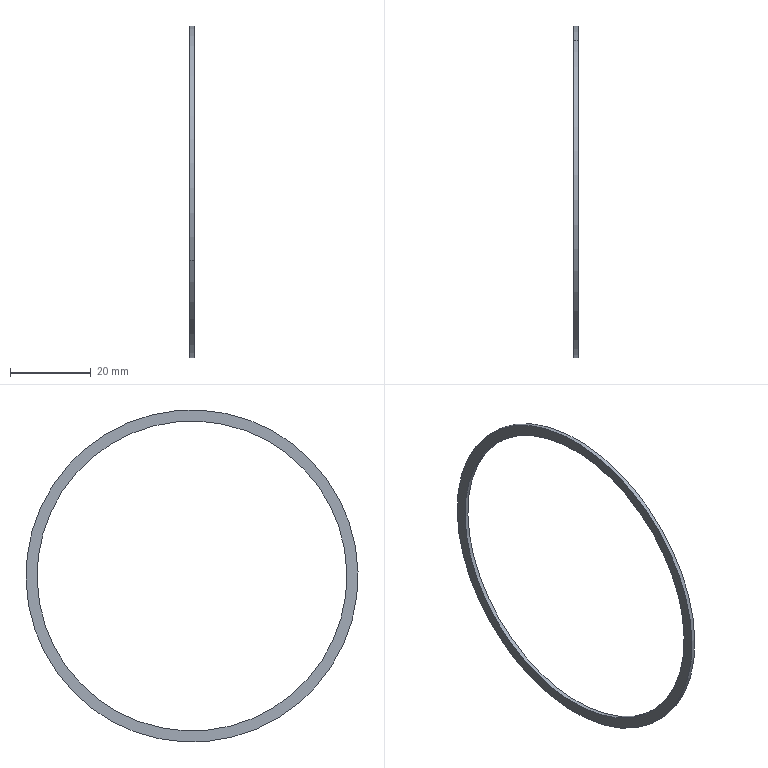Component | SolidWorks | 2018SOLIDWORKS1000000503-1 | 1 solid | 6 faces | box 1 x 82 x 82 mm | volume 685 mm3 | cylinder 4 | plane 2 | commonest cylinder face diameters 76.5 x2 82 x2 | material 201
build123d program:
from build123d import *

# Parameters (mm, degrees)
SKETCH1_R           = 41
SKETCH1_R_2         = 38.25
BOSS_EXTRUDE1_DEPTH = 1


with BuildPart() as part:
    # Sketch1 → Boss-Extrude1 (new body)
    with BuildSketch(Plane.XY):
        Circle(SKETCH1_R)
        Circle(SKETCH1_R_2, mode=Mode.SUBTRACT)
    extrude(amount=BOSS_EXTRUDE1_DEPTH)


solid = part.part

# Placed as in the assembly
solid = solid.moved(Location((6.716, -95.825, 207.018), (0, 90, 0)))
STEP:
#1=COLOUR_RGB('',0.7922,0.8196,0.9333);
#2=FILL_AREA_STYLE_COLOUR('',#1);
#3=FILL_AREA_STYLE('',(#2));
#4=SURFACE_STYLE_FILL_AREA(#3);
#5=SURFACE_SIDE_STYLE('',(#4));
#6=SURFACE_STYLE_USAGE(.BOTH.,#5);
#7=PRESENTATION_STYLE_ASSIGNMENT((#6));
#8=CARTESIAN_POINT('',(0.3038,-5.145,7.53));
#9=VERTEX_POINT('',#8);
#10=CARTESIAN_POINT('',(0.3038,-2.4,8.771));
#11=VERTEX_POINT('',#10);
#12=CARTESIAN_POINT('',(0.3038,-3.773,8.15));
#13=DIRECTION('',(1.,0.,-0.));
#14=DIRECTION('',(-0.,0.9112,0.4119));
#15=AXIS2_PLACEMENT_3D('',#12,#13,#14);
#16=CIRCLE('',#15,1.506);
#17=EDGE_CURVE('',#9,#11,#16,.T.);
#18=ORIENTED_EDGE('',*,*,#17,.T.);
#19=CARTESIAN_POINT('',(0.2644,-2.4,8.771));
#20=VERTEX_POINT('',#19);
#21=CARTESIAN_POINT('',(0.3038,-2.4,8.771));
#22=DIRECTION('',(-1.,-0.,0.));
#23=VECTOR('',#22,39.37);
#24=LINE('',#21,#23);
#25=EDGE_CURVE('',#11,#20,#24,.T.);
#26=ORIENTED_EDGE('',*,*,#25,.T.);
#27=CARTESIAN_POINT('',(0.2644,-5.145,7.53));
#28=VERTEX_POINT('',#27);
#29=CARTESIAN_POINT('',(0.2644,-3.773,8.15));
#30=DIRECTION('',(1.,0.,-0.));
#31=DIRECTION('',(-0.,0.9112,0.4119));
#32=AXIS2_PLACEMENT_3D('',#29,#30,#31);
#33=CIRCLE('',#32,1.506);
#34=EDGE_CURVE('',#28,#20,#33,.T.);
#35=ORIENTED_EDGE('',*,*,#34,.F.);
#36=CARTESIAN_POINT('',(0.3038,-5.145,7.53));
#37=DIRECTION('',(-1.,-0.,0.));
#38=VECTOR('',#37,39.37);
#39=LINE('',#36,#38);
#40=EDGE_CURVE('',#9,#28,#39,.T.);
#41=ORIENTED_EDGE('',*,*,#40,.F.);
#42=EDGE_LOOP('',(#18,#26,#35,#41));
#43=FACE_OUTER_BOUND('',#42,.T.);
#44=CARTESIAN_POINT('',(0.3038,-3.773,8.15));
#45=DIRECTION('',(-1.,-0.,0.));
#46=DIRECTION('',(0.,-0.9112,-0.4119));
#47=AXIS2_PLACEMENT_3D('',#44,#45,#46);
#48=CYLINDRICAL_SURFACE('',#47,1.506);
#49=ADVANCED_FACE('',(#43),#48,.F.);
#50=CARTESIAN_POINT('',(0.3038,-2.302,8.815));
#51=VERTEX_POINT('',#50);
#52=CARTESIAN_POINT('',(0.3038,-5.244,7.485));
#53=VERTEX_POINT('',#52);
#54=CARTESIAN_POINT('',(0.3038,-3.773,8.15));
#55=DIRECTION('',(1.,0.,-0.));
#56=DIRECTION('',(-0.,0.9112,0.4119));
#57=AXIS2_PLACEMENT_3D('',#54,#55,#56);
#58=CIRCLE('',#57,1.614);
#59=EDGE_CURVE('',#51,#53,#58,.T.);
#60=ORIENTED_EDGE('',*,*,#59,.F.);
#61=CARTESIAN_POINT('',(0.2644,-2.302,8.815));
#62=VERTEX_POINT('',#61);
#63=CARTESIAN_POINT('',(0.3038,-2.302,8.815));
#64=DIRECTION('',(-1.,-0.,0.));
#65=VECTOR('',#64,39.37);
#66=LINE('',#63,#65);
#67=EDGE_CURVE('',#51,#62,#66,.T.);
#68=ORIENTED_EDGE('',*,*,#67,.T.);
#69=CARTESIAN_POINT('',(0.2644,-5.244,7.485));
#70=VERTEX_POINT('',#69);
#71=CARTESIAN_POINT('',(0.2644,-3.773,8.15));
#72=DIRECTION('',(1.,0.,-0.));
#73=DIRECTION('',(-0.,0.9112,0.4119));
#74=AXIS2_PLACEMENT_3D('',#71,#72,#73);
#75=CIRCLE('',#74,1.614);
#76=EDGE_CURVE('',#62,#70,#75,.T.);
#77=ORIENTED_EDGE('',*,*,#76,.T.);
#78=CARTESIAN_POINT('',(0.3038,-5.244,7.485));
#79=DIRECTION('',(-1.,-0.,0.));
#80=VECTOR('',#79,39.37);
#81=LINE('',#78,#80);
#82=EDGE_CURVE('',#53,#70,#81,.T.);
#83=ORIENTED_EDGE('',*,*,#82,.F.);
#84=EDGE_LOOP('',(#60,#68,#77,#83));
#85=FACE_OUTER_BOUND('',#84,.T.);
#86=CARTESIAN_POINT('',(0.3038,-3.773,8.15));
#87=DIRECTION('',(-1.,-0.,0.));
#88=DIRECTION('',(0.,-0.9112,-0.4119));
#89=AXIS2_PLACEMENT_3D('',#86,#87,#88);
#90=CYLINDRICAL_SURFACE('',#89,1.614);
#91=ADVANCED_FACE('',(#85),#90,.T.);
#92=CARTESIAN_POINT('',(0.3038,-3.773,8.15));
#93=DIRECTION('',(1.,0.,-0.));
#94=DIRECTION('',(-0.,0.9112,0.4119));
#95=AXIS2_PLACEMENT_3D('',#92,#93,#94);
#96=CIRCLE('',#95,1.614);
#97=EDGE_CURVE('',#53,#51,#96,.T.);
#98=ORIENTED_EDGE('',*,*,#97,.T.);
#99=ORIENTED_EDGE('',*,*,#59,.T.);
#100=EDGE_LOOP('',(#98,#99));
#101=FACE_OUTER_BOUND('',#100,.T.);
#102=ORIENTED_EDGE('',*,*,#17,.F.);
#103=CARTESIAN_POINT('',(0.3038,-3.773,8.15));
#104=DIRECTION('',(1.,0.,-0.));
#105=DIRECTION('',(-0.,0.9112,0.4119));
#106=AXIS2_PLACEMENT_3D('',#103,#104,#105);
#107=CIRCLE('',#106,1.506);
#108=EDGE_CURVE('',#11,#9,#107,.T.);
#109=ORIENTED_EDGE('',*,*,#108,.F.);
#110=EDGE_LOOP('',(#102,#109));
#111=FACE_BOUND('',#110,.T.);
#112=CARTESIAN_POINT('',(0.3038,-3.773,8.15));
#113=DIRECTION('',(1.,0.,-0.));
#114=DIRECTION('',(-0.,0.9112,0.4119));
#115=AXIS2_PLACEMENT_3D('',#112,#113,#114);
#116=PLANE('',#115);
#117=ADVANCED_FACE('',(#101,#111),#116,.T.);
#118=CARTESIAN_POINT('',(0.2644,-3.773,8.15));
#119=DIRECTION('',(1.,0.,-0.));
#120=DIRECTION('',(-0.,0.9112,0.4119));
#121=AXIS2_PLACEMENT_3D('',#118,#119,#120);
#122=CIRCLE('',#121,1.614);
#123=EDGE_CURVE('',#70,#62,#122,.T.);
#124=ORIENTED_EDGE('',*,*,#123,.F.);
#125=ORIENTED_EDGE('',*,*,#76,.F.);
#126=EDGE_LOOP('',(#124,#125));
#127=FACE_OUTER_BOUND('',#126,.T.);
#128=ORIENTED_EDGE('',*,*,#34,.T.);
#129=CARTESIAN_POINT('',(0.2644,-3.773,8.15));
#130=DIRECTION('',(1.,0.,-0.));
#131=DIRECTION('',(-0.,0.9112,0.4119));
#132=AXIS2_PLACEMENT_3D('',#129,#130,#131);
#133=CIRCLE('',#132,1.506);
#134=EDGE_CURVE('',#20,#28,#133,.T.);
#135=ORIENTED_EDGE('',*,*,#134,.T.);
#136=EDGE_LOOP('',(#128,#135));
#137=FACE_BOUND('',#136,.T.);
#138=CARTESIAN_POINT('',(0.2644,-3.773,8.15));
#139=DIRECTION('',(1.,0.,-0.));
#140=DIRECTION('',(-0.,0.9112,0.4119));
#141=AXIS2_PLACEMENT_3D('',#138,#139,#140);
#142=PLANE('',#141);
#143=ADVANCED_FACE('',(#127,#137),#142,.F.);
#144=ORIENTED_EDGE('',*,*,#67,.F.);
#145=ORIENTED_EDGE('',*,*,#97,.F.);
#146=ORIENTED_EDGE('',*,*,#82,.T.);
#147=ORIENTED_EDGE('',*,*,#123,.T.);
#148=EDGE_LOOP('',(#144,#145,#146,#147));
#149=FACE_OUTER_BOUND('',#148,.T.);
#150=CARTESIAN_POINT('',(0.3038,-3.773,8.15));
#151=DIRECTION('',(-1.,-0.,0.));
#152=DIRECTION('',(0.,-0.9112,-0.4119));
#153=AXIS2_PLACEMENT_3D('',#150,#151,#152);
#154=CYLINDRICAL_SURFACE('',#153,1.614);
#155=ADVANCED_FACE('',(#149),#154,.T.);
#156=ORIENTED_EDGE('',*,*,#25,.F.);
#157=ORIENTED_EDGE('',*,*,#108,.T.);
#158=ORIENTED_EDGE('',*,*,#40,.T.);
#159=ORIENTED_EDGE('',*,*,#134,.F.);
#160=EDGE_LOOP('',(#156,#157,#158,#159));
#161=FACE_OUTER_BOUND('',#160,.T.);
#162=CARTESIAN_POINT('',(0.3038,-3.773,8.15));
#163=DIRECTION('',(-1.,-0.,0.));
#164=DIRECTION('',(0.,-0.9112,-0.4119));
#165=AXIS2_PLACEMENT_3D('',#162,#163,#164);
#166=CYLINDRICAL_SURFACE('',#165,1.506);
#167=ADVANCED_FACE('',(#161),#166,.F.);
#168=CLOSED_SHELL('',(#49,#91,#117,#143,#155,#167));
#169=MANIFOLD_SOLID_BREP('',#168);
#170=STYLED_ITEM('',(#7),#169);
#171=PRESENTATION_LAYER_ASSIGNMENT('','',(#170));
#172=(LENGTH_UNIT()NAMED_UNIT(*)SI_UNIT($,.METRE.));
#173=LENGTH_MEASURE_WITH_UNIT(LENGTH_MEASURE(0.0254),#172);
#174=DIMENSIONAL_EXPONENTS(1.,0.,0.,0.,0.,0.,0.);
#175=(CONVERSION_BASED_UNIT('',#173)LENGTH_UNIT()NAMED_UNIT(#174));
#176=UNCERTAINTY_MEASURE_WITH_UNIT(LENGTH_MEASURE(0.00001),#175,'','');
#177=(NAMED_UNIT(*)PLANE_ANGLE_UNIT()SI_UNIT($,.RADIAN.));
#178=(NAMED_UNIT(*)SI_UNIT($,.STERADIAN.)SOLID_ANGLE_UNIT());
#179=(GEOMETRIC_REPRESENTATION_CONTEXT(3)GLOBAL_UNCERTAINTY_ASSIGNED_CONTEXT((#176))GLOBAL_UNIT_ASSIGNED_CONTEXT((#175,#177,#178))REPRESENTATION_CONTEXT('',''));
#180=MECHANICAL_DESIGN_GEOMETRIC_PRESENTATION_REPRESENTATION('',(#170),#179);
#181=CARTESIAN_POINT('',(0.,0.,0.));
#182=DIRECTION('',(0.,0.,1.));
#183=DIRECTION('',(1.,0.,0.));
#184=AXIS2_PLACEMENT_3D('',#181,#182,#183);
#185=(LENGTH_UNIT()NAMED_UNIT(*)SI_UNIT($,.METRE.));
#186=LENGTH_MEASURE_WITH_UNIT(LENGTH_MEASURE(0.0254),#185);
#187=DIMENSIONAL_EXPONENTS(1.,0.,0.,0.,0.,0.,0.);
#188=(CONVERSION_BASED_UNIT('',#186)LENGTH_UNIT()NAMED_UNIT(#187));
#189=UNCERTAINTY_MEASURE_WITH_UNIT(LENGTH_MEASURE(0.00001),#188,'','');
#190=(NAMED_UNIT(*)PLANE_ANGLE_UNIT()SI_UNIT($,.RADIAN.));
#191=(NAMED_UNIT(*)SI_UNIT($,.STERADIAN.)SOLID_ANGLE_UNIT());
#192=(GEOMETRIC_REPRESENTATION_CONTEXT(3)GLOBAL_UNCERTAINTY_ASSIGNED_CONTEXT((#189))GLOBAL_UNIT_ASSIGNED_CONTEXT((#188,#190,#191))REPRESENTATION_CONTEXT('',''));
#193=ADVANCED_BREP_SHAPE_REPRESENTATION('',(#169,#184),#192);